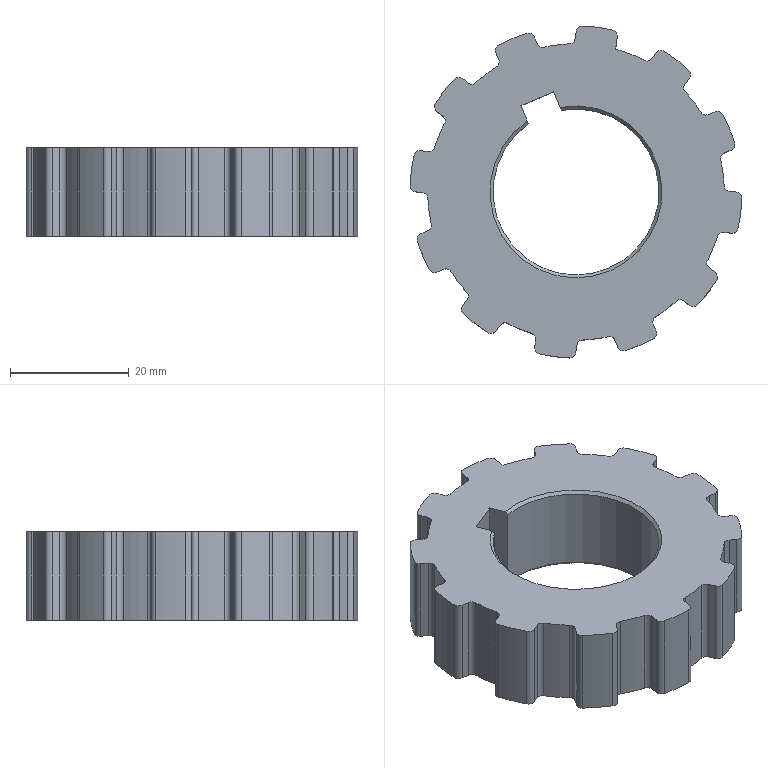Component | NX | RATCHET | 1 solid | 103 faces | volume 23696 mm3 | cylinder 72 | plane 29 | cone 2 | commonest cylinder face diameters 2 x47 56 x12 50 x12 28 x1